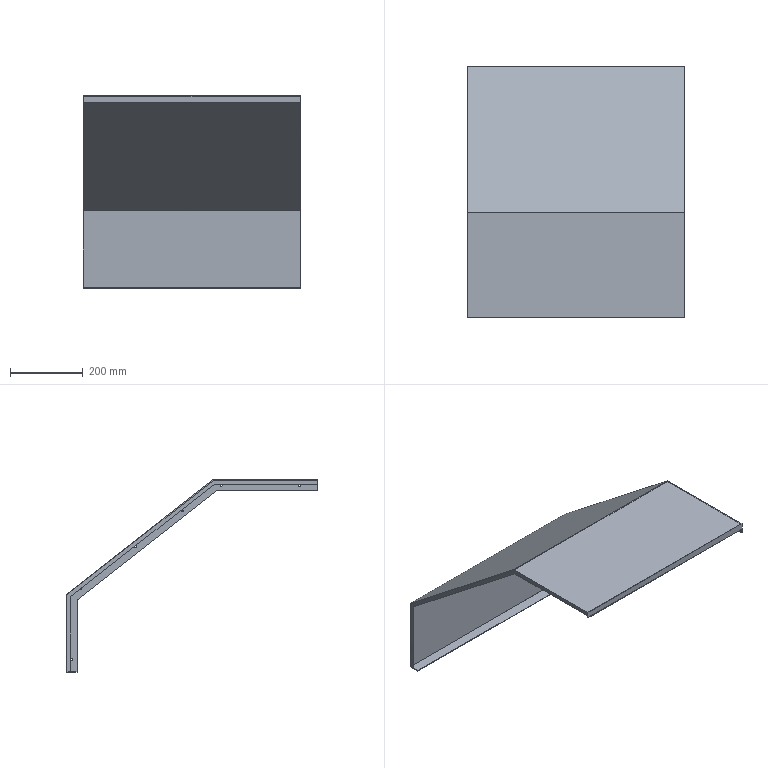Component | SolidWorks | FrontBaffle-1 | 1 solid | 33 faces | box 597 x 690 x 527.05 mm | volume 1332311 mm3 | plane 21 | cylinder 12 | commonest cylinder face diameters 6 x12
build123d program:
from build123d import *

# Parameters (mm, degrees)
EXTRUDE_THIN1_DEPTH = 595
SHELL1_T            = -2
EXTRUDE_THIN2_DEPTH = 2
SKETCH3_W           = 597
SKETCH3_H           = 2
EXTRUDE_THIN3_DEPTH = 16
SKETCH4_W           = 597
SKETCH4_H           = 30
BOSS_EXTRUDE1_DEPTH = 2
SKETCH5_R           = 3
CUT_EXTRUDE1_DEPTH  = 2


with BuildPart() as part:
    # Sketch1 → Extrude-Thin1 (new body)
    with BuildSketch(Plane.XY):
        Polygon((-90.472, -281.746), (-90.472, 6.2), (223.646, 408.252), (436.576, 408.252), (436.576, 378.252), (238.278, 378.252), (-60.472, -4.13), (-60.472, -281.746), align=None)
    extrude(amount=EXTRUDE_THIN1_DEPTH)

    # Shell1
    shell1_openings = [part.faces().sort_by_distance(p)[0] for p in [
        (88.903, 187.061, 297.5),
        (-60.472, -142.938, 297.5),
        (-75.472, -281.746, 297.5),
        (436.576, 393.252, 297.5),
        (337.427, 378.252, 297.5),
        (-81.789, -137.773, 0),
    ]]
    offset(amount=SHELL1_T, openings=shell1_openings, kind=Kind.INTERSECTION)

    # Sketch2 → Extrude-Thin2 (add)
    with BuildSketch(Plane(origin=(0, 0, 0), x_dir=(-1, 0, 0), z_dir=(0, 0, -1))):
        Polygon((-436.576, 408.252), (-223.646, 408.252), (90.472, 6.2), (90.472, -281.746), (78.472, -281.746), (78.472, 2.068), (-229.499, 396.252), (-436.576, 396.252), align=None)
    extrude(amount=EXTRUDE_THIN2_DEPTH)

    # Sketch3 → Extrude-Thin3 (add)
    with BuildSketch(Plane(origin=(-88.472, 0, 0), x_dir=(0, 0, -1), z_dir=(1, 0, 0))):
        with Locations((-296.5, -280.746)):
            Rectangle(SKETCH3_W, SKETCH3_H)
    extrude(amount=EXTRUDE_THIN3_DEPTH)

    # Sketch4 → Boss-Extrude1 (add)
    with BuildSketch(Plane(origin=(436.576, 0, 0), x_dir=(0, 0, -1), z_dir=(1, 0, 0))):
        with Locations((-296.5, 393.252)):
            Rectangle(SKETCH4_W, SKETCH4_H)
    extrude(amount=-BOSS_EXTRUDE1_DEPTH)

    # Sketch5 → Cut-Extrude1 (cut)
    with BuildSketch(Plane.XY.offset(595)):
        with Locations((-75.472, -231.746)):
            Circle(SKETCH5_R)
        with Locations((-75.472, -16.746)):
            Circle(SKETCH5_R)
        with Locations((-5.552, 90.528)):
            Circle(SKETCH5_R)
        with Locations((92.065, 217.3)):
            Circle(SKETCH5_R)
        with Locations((207.86, 367.937)):
            Circle(SKETCH5_R)
        with Locations((401.576, 393.252)):
            Circle(SKETCH5_R)
    extrude(amount=-CUT_EXTRUDE1_DEPTH, mode=Mode.SUBTRACT)


solid = part.part

# Placed as in the assembly
solid = solid.moved(Location((-889.55, -36.686, 386.009), (0, 90, 0)))
STEP:
#1=COLOUR_RGB('',0.7922,0.8196,0.9333);
#2=FILL_AREA_STYLE_COLOUR('',#1);
#3=FILL_AREA_STYLE('',(#2));
#4=SURFACE_STYLE_FILL_AREA(#3);
#5=SURFACE_SIDE_STYLE('',(#4));
#6=SURFACE_STYLE_USAGE(.BOTH.,#5);
#7=PRESENTATION_STYLE_ASSIGNMENT((#6));
#8=CARTESIAN_POINT('',(-11.675,14.038,-0.4948));
#9=VERTEX_POINT('',#8);
#10=CARTESIAN_POINT('',(-11.675,14.038,-0.731));
#11=VERTEX_POINT('',#10);
#12=CARTESIAN_POINT('',(-11.675,14.038,-0.6129));
#13=DIRECTION('',(1.,0.,-0.));
#14=DIRECTION('',(0.,0.,-1.));
#15=AXIS2_PLACEMENT_3D('',#12,#13,#14);
#16=CIRCLE('',#15,0.1181);
#17=EDGE_CURVE('',#9,#11,#16,.T.);
#18=ORIENTED_EDGE('',*,*,#17,.F.);
#19=CARTESIAN_POINT('',(-11.596,14.038,-0.4948));
#20=VERTEX_POINT('',#19);
#21=CARTESIAN_POINT('',(-11.675,14.038,-0.4948));
#22=DIRECTION('',(1.,0.,-0.));
#23=VECTOR('',#22,39.37);
#24=LINE('',#21,#23);
#25=EDGE_CURVE('',#9,#20,#24,.T.);
#26=ORIENTED_EDGE('',*,*,#25,.T.);
#27=CARTESIAN_POINT('',(-11.596,14.038,-0.731));
#28=VERTEX_POINT('',#27);
#29=CARTESIAN_POINT('',(-11.596,14.038,-0.6129));
#30=DIRECTION('',(1.,0.,-0.));
#31=DIRECTION('',(0.,0.,-1.));
#32=AXIS2_PLACEMENT_3D('',#29,#30,#31);
#33=CIRCLE('',#32,0.1181);
#34=EDGE_CURVE('',#20,#28,#33,.T.);
#35=ORIENTED_EDGE('',*,*,#34,.T.);
#36=CARTESIAN_POINT('',(-11.675,14.038,-0.731));
#37=DIRECTION('',(1.,0.,-0.));
#38=VECTOR('',#37,39.37);
#39=LINE('',#36,#38);
#40=EDGE_CURVE('',#11,#28,#39,.T.);
#41=ORIENTED_EDGE('',*,*,#40,.F.);
#42=EDGE_LOOP('',(#18,#26,#35,#41));
#43=FACE_OUTER_BOUND('',#42,.T.);
#44=CARTESIAN_POINT('',(-11.675,14.038,-0.6129));
#45=DIRECTION('',(1.,0.,-0.));
#46=DIRECTION('',(0.,0.,-1.));
#47=AXIS2_PLACEMENT_3D('',#44,#45,#46);
#48=CYLINDRICAL_SURFACE('',#47,0.1181);
#49=ADVANCED_FACE('',(#43),#48,.F.);
#50=CARTESIAN_POINT('',(-11.675,13.041,7.132));
#51=VERTEX_POINT('',#50);
#52=CARTESIAN_POINT('',(-11.675,13.041,6.896));
#53=VERTEX_POINT('',#52);
#54=CARTESIAN_POINT('',(-11.675,13.041,7.014));
#55=DIRECTION('',(1.,0.,-0.));
#56=DIRECTION('',(0.,0.,-1.));
#57=AXIS2_PLACEMENT_3D('',#54,#55,#56);
#58=CIRCLE('',#57,0.1181);
#59=EDGE_CURVE('',#51,#53,#58,.T.);
#60=ORIENTED_EDGE('',*,*,#59,.F.);
#61=CARTESIAN_POINT('',(-11.596,13.041,7.132));
#62=VERTEX_POINT('',#61);
#63=CARTESIAN_POINT('',(-11.675,13.041,7.132));
#64=DIRECTION('',(1.,0.,-0.));
#65=VECTOR('',#64,39.37);
#66=LINE('',#63,#65);
#67=EDGE_CURVE('',#51,#62,#66,.T.);
#68=ORIENTED_EDGE('',*,*,#67,.T.);
#69=CARTESIAN_POINT('',(-11.596,13.041,6.896));
#70=VERTEX_POINT('',#69);
#71=CARTESIAN_POINT('',(-11.596,13.041,7.014));
#72=DIRECTION('',(1.,0.,-0.));
#73=DIRECTION('',(0.,0.,-1.));
#74=AXIS2_PLACEMENT_3D('',#71,#72,#73);
#75=CIRCLE('',#74,0.1181);
#76=EDGE_CURVE('',#62,#70,#75,.T.);
#77=ORIENTED_EDGE('',*,*,#76,.T.);
#78=CARTESIAN_POINT('',(-11.675,13.041,6.896));
#79=DIRECTION('',(1.,0.,-0.));
#80=VECTOR('',#79,39.37);
#81=LINE('',#78,#80);
#82=EDGE_CURVE('',#53,#70,#81,.T.);
#83=ORIENTED_EDGE('',*,*,#82,.F.);
#84=EDGE_LOOP('',(#60,#68,#77,#83));
#85=FACE_OUTER_BOUND('',#84,.T.);
#86=CARTESIAN_POINT('',(-11.675,13.041,7.014));
#87=DIRECTION('',(1.,0.,-0.));
#88=DIRECTION('',(0.,0.,-1.));
#89=AXIS2_PLACEMENT_3D('',#86,#87,#88);
#90=CYLINDRICAL_SURFACE('',#89,0.1181);
#91=ADVANCED_FACE('',(#85),#90,.F.);
#92=CARTESIAN_POINT('',(-11.675,7.111,11.691));
#93=VERTEX_POINT('',#92);
#94=CARTESIAN_POINT('',(-11.675,7.111,11.455));
#95=VERTEX_POINT('',#94);
#96=CARTESIAN_POINT('',(-11.675,7.111,11.573));
#97=DIRECTION('',(1.,0.,-0.));
#98=DIRECTION('',(0.,0.,-1.));
#99=AXIS2_PLACEMENT_3D('',#96,#97,#98);
#100=CIRCLE('',#99,0.1181);
#101=EDGE_CURVE('',#93,#95,#100,.T.);
#102=ORIENTED_EDGE('',*,*,#101,.F.);
#103=CARTESIAN_POINT('',(-11.596,7.111,11.691));
#104=VERTEX_POINT('',#103);
#105=CARTESIAN_POINT('',(-11.675,7.111,11.691));
#106=DIRECTION('',(1.,0.,-0.));
#107=VECTOR('',#106,39.37);
#108=LINE('',#105,#107);
#109=EDGE_CURVE('',#93,#104,#108,.T.);
#110=ORIENTED_EDGE('',*,*,#109,.T.);
#111=CARTESIAN_POINT('',(-11.596,7.111,11.455));
#112=VERTEX_POINT('',#111);
#113=CARTESIAN_POINT('',(-11.596,7.111,11.573));
#114=DIRECTION('',(1.,0.,-0.));
#115=DIRECTION('',(0.,0.,-1.));
#116=AXIS2_PLACEMENT_3D('',#113,#114,#115);
#117=CIRCLE('',#116,0.1181);
#118=EDGE_CURVE('',#104,#112,#117,.T.);
#119=ORIENTED_EDGE('',*,*,#118,.T.);
#120=CARTESIAN_POINT('',(-11.675,7.111,11.455));
#121=DIRECTION('',(1.,0.,-0.));
#122=VECTOR('',#121,39.37);
#123=LINE('',#120,#122);
#124=EDGE_CURVE('',#95,#112,#123,.T.);
#125=ORIENTED_EDGE('',*,*,#124,.F.);
#126=EDGE_LOOP('',(#102,#110,#119,#125));
#127=FACE_OUTER_BOUND('',#126,.T.);
#128=CARTESIAN_POINT('',(-11.675,7.111,11.573));
#129=DIRECTION('',(1.,0.,-0.));
#130=DIRECTION('',(0.,0.,-1.));
#131=AXIS2_PLACEMENT_3D('',#128,#129,#130);
#132=CYLINDRICAL_SURFACE('',#131,0.1181);
#133=ADVANCED_FACE('',(#127),#132,.F.);
#134=CARTESIAN_POINT('',(-11.675,2.12,15.534));
#135=VERTEX_POINT('',#134);
#136=CARTESIAN_POINT('',(-11.675,2.12,15.298));
#137=VERTEX_POINT('',#136);
#138=CARTESIAN_POINT('',(-11.675,2.12,15.416));
#139=DIRECTION('',(1.,0.,-0.));
#140=DIRECTION('',(0.,0.,-1.));
#141=AXIS2_PLACEMENT_3D('',#138,#139,#140);
#142=CIRCLE('',#141,0.1181);
#143=EDGE_CURVE('',#135,#137,#142,.T.);
#144=ORIENTED_EDGE('',*,*,#143,.F.);
#145=CARTESIAN_POINT('',(-11.596,2.12,15.534));
#146=VERTEX_POINT('',#145);
#147=CARTESIAN_POINT('',(-11.675,2.12,15.534));
#148=DIRECTION('',(1.,0.,-0.));
#149=VECTOR('',#148,39.37);
#150=LINE('',#147,#149);
#151=EDGE_CURVE('',#135,#146,#150,.T.);
#152=ORIENTED_EDGE('',*,*,#151,.T.);
#153=CARTESIAN_POINT('',(-11.596,2.12,15.298));
#154=VERTEX_POINT('',#153);
#155=CARTESIAN_POINT('',(-11.596,2.12,15.416));
#156=DIRECTION('',(1.,0.,-0.));
#157=DIRECTION('',(0.,0.,-1.));
#158=AXIS2_PLACEMENT_3D('',#155,#156,#157);
#159=CIRCLE('',#158,0.1181);
#160=EDGE_CURVE('',#146,#154,#159,.T.);
#161=ORIENTED_EDGE('',*,*,#160,.T.);
#162=CARTESIAN_POINT('',(-11.675,2.12,15.298));
#163=DIRECTION('',(1.,0.,-0.));
#164=VECTOR('',#163,39.37);
#165=LINE('',#162,#164);
#166=EDGE_CURVE('',#137,#154,#165,.T.);
#167=ORIENTED_EDGE('',*,*,#166,.F.);
#168=EDGE_LOOP('',(#144,#152,#161,#167));
#169=FACE_OUTER_BOUND('',#168,.T.);
#170=CARTESIAN_POINT('',(-11.675,2.12,15.416));
#171=DIRECTION('',(1.,0.,-0.));
#172=DIRECTION('',(0.,0.,-1.));
#173=AXIS2_PLACEMENT_3D('',#170,#171,#172);
#174=CYLINDRICAL_SURFACE('',#173,0.1181);
#175=ADVANCED_FACE('',(#169),#174,.F.);
#176=CARTESIAN_POINT('',(-11.675,-2.104,18.287));
#177=VERTEX_POINT('',#176);
#178=CARTESIAN_POINT('',(-11.675,-2.104,18.05));
#179=VERTEX_POINT('',#178);
#180=CARTESIAN_POINT('',(-11.675,-2.104,18.169));
#181=DIRECTION('',(1.,0.,-0.));
#182=DIRECTION('',(0.,0.,-1.));
#183=AXIS2_PLACEMENT_3D('',#180,#181,#182);
#184=CIRCLE('',#183,0.1181);
#185=EDGE_CURVE('',#177,#179,#184,.T.);
#186=ORIENTED_EDGE('',*,*,#185,.F.);
#187=CARTESIAN_POINT('',(-11.596,-2.104,18.287));
#188=VERTEX_POINT('',#187);
#189=CARTESIAN_POINT('',(-11.675,-2.104,18.287));
#190=DIRECTION('',(1.,0.,-0.));
#191=VECTOR('',#190,39.37);
#192=LINE('',#189,#191);
#193=EDGE_CURVE('',#177,#188,#192,.T.);
#194=ORIENTED_EDGE('',*,*,#193,.T.);
#195=CARTESIAN_POINT('',(-11.596,-2.104,18.05));
#196=VERTEX_POINT('',#195);
#197=CARTESIAN_POINT('',(-11.596,-2.104,18.169));
#198=DIRECTION('',(1.,0.,-0.));
#199=DIRECTION('',(0.,0.,-1.));
#200=AXIS2_PLACEMENT_3D('',#197,#198,#199);
#201=CIRCLE('',#200,0.1181);
#202=EDGE_CURVE('',#188,#196,#201,.T.);
#203=ORIENTED_EDGE('',*,*,#202,.T.);
#204=CARTESIAN_POINT('',(-11.675,-2.104,18.05));
#205=DIRECTION('',(1.,0.,-0.));
#206=VECTOR('',#205,39.37);
#207=LINE('',#204,#206);
#208=EDGE_CURVE('',#179,#196,#207,.T.);
#209=ORIENTED_EDGE('',*,*,#208,.F.);
#210=EDGE_LOOP('',(#186,#194,#203,#209));
#211=FACE_OUTER_BOUND('',#210,.T.);
#212=CARTESIAN_POINT('',(-11.675,-2.104,18.169));
#213=DIRECTION('',(1.,0.,-0.));
#214=DIRECTION('',(0.,0.,-1.));
#215=AXIS2_PLACEMENT_3D('',#212,#213,#214);
#216=CYLINDRICAL_SURFACE('',#215,0.1181);
#217=ADVANCED_FACE('',(#211),#216,.F.);
#218=CARTESIAN_POINT('',(-11.675,-10.568,18.287));
#219=VERTEX_POINT('',#218);
#220=CARTESIAN_POINT('',(-11.675,-10.568,18.05));
#221=VERTEX_POINT('',#220);
#222=CARTESIAN_POINT('',(-11.675,-10.568,18.169));
#223=DIRECTION('',(1.,0.,-0.));
#224=DIRECTION('',(0.,0.,-1.));
#225=AXIS2_PLACEMENT_3D('',#222,#223,#224);
#226=CIRCLE('',#225,0.1181);
#227=EDGE_CURVE('',#219,#221,#226,.T.);
#228=ORIENTED_EDGE('',*,*,#227,.F.);
#229=CARTESIAN_POINT('',(-11.596,-10.568,18.287));
#230=VERTEX_POINT('',#229);
#231=CARTESIAN_POINT('',(-11.675,-10.568,18.287));
#232=DIRECTION('',(1.,0.,-0.));
#233=VECTOR('',#232,39.37);
#234=LINE('',#231,#233);
#235=EDGE_CURVE('',#219,#230,#234,.T.);
#236=ORIENTED_EDGE('',*,*,#235,.T.);
#237=CARTESIAN_POINT('',(-11.596,-10.568,18.05));
#238=VERTEX_POINT('',#237);
#239=CARTESIAN_POINT('',(-11.596,-10.568,18.169));
#240=DIRECTION('',(1.,0.,-0.));
#241=DIRECTION('',(0.,0.,-1.));
#242=AXIS2_PLACEMENT_3D('',#239,#240,#241);
#243=CIRCLE('',#242,0.1181);
#244=EDGE_CURVE('',#230,#238,#243,.T.);
#245=ORIENTED_EDGE('',*,*,#244,.T.);
#246=CARTESIAN_POINT('',(-11.675,-10.568,18.05));
#247=DIRECTION('',(1.,0.,-0.));
#248=VECTOR('',#247,39.37);
#249=LINE('',#246,#248);
#250=EDGE_CURVE('',#221,#238,#249,.T.);
#251=ORIENTED_EDGE('',*,*,#250,.F.);
#252=EDGE_LOOP('',(#228,#236,#245,#251));
#253=FACE_OUTER_BOUND('',#252,.T.);
#254=CARTESIAN_POINT('',(-11.675,-10.568,18.169));
#255=DIRECTION('',(1.,0.,-0.));
#256=DIRECTION('',(0.,0.,-1.));
#257=AXIS2_PLACEMENT_3D('',#254,#255,#256);
#258=CYLINDRICAL_SURFACE('',#257,0.1181);
#259=ADVANCED_FACE('',(#253),#258,.F.);
#260=CARTESIAN_POINT('',(-11.675,14.55,-1.912));
#261=VERTEX_POINT('',#260);
#262=CARTESIAN_POINT('',(-35.022,14.55,-1.912));
#263=VERTEX_POINT('',#262);
#264=CARTESIAN_POINT('',(-11.596,14.55,-1.912));
#265=DIRECTION('',(-1.,-0.,0.));
#266=VECTOR('',#265,39.37);
#267=LINE('',#264,#266);
#268=EDGE_CURVE('',#261,#263,#267,.T.);
#269=ORIENTED_EDGE('',*,*,#268,.F.);
#270=CARTESIAN_POINT('',(-11.675,14.55,6.354));
#271=VERTEX_POINT('',#270);
#272=CARTESIAN_POINT('',(-11.675,14.55,15.197));
#273=DIRECTION('',(-0.,-0.,-1.));
#274=VECTOR('',#273,39.37);
#275=LINE('',#272,#274);
#276=EDGE_CURVE('',#271,#261,#275,.T.);
#277=ORIENTED_EDGE('',*,*,#276,.F.);
#278=CARTESIAN_POINT('',(-35.022,14.55,6.354));
#279=VERTEX_POINT('',#278);
#280=CARTESIAN_POINT('',(-11.596,14.55,6.354));
#281=DIRECTION('',(-1.,-0.,0.));
#282=VECTOR('',#281,39.37);
#283=LINE('',#280,#282);
#284=EDGE_CURVE('',#271,#279,#283,.T.);
#285=ORIENTED_EDGE('',*,*,#284,.T.);
#286=CARTESIAN_POINT('',(-35.022,14.55,15.197));
#287=DIRECTION('',(-0.,-0.,-1.));
#288=VECTOR('',#287,39.37);
#289=LINE('',#286,#288);
#290=EDGE_CURVE('',#279,#263,#289,.T.);
#291=ORIENTED_EDGE('',*,*,#290,.T.);
#292=EDGE_LOOP('',(#269,#277,#285,#291));
#293=FACE_OUTER_BOUND('',#292,.T.);
#294=CARTESIAN_POINT('',(-11.596,14.55,6.392));
#295=DIRECTION('',(-0.,1.,-0.));
#296=DIRECTION('',(0.,0.,1.));
#297=AXIS2_PLACEMENT_3D('',#294,#295,#296);
#298=PLANE('',#297);
#299=ADVANCED_FACE('',(#293),#298,.F.);
#300=CARTESIAN_POINT('',(-11.675,14.038,-0.6129));
#301=DIRECTION('',(1.,0.,-0.));
#302=DIRECTION('',(0.,0.,-1.));
#303=AXIS2_PLACEMENT_3D('',#300,#301,#302);
#304=CIRCLE('',#303,0.1181);
#305=EDGE_CURVE('',#11,#9,#304,.T.);
#306=ORIENTED_EDGE('',*,*,#305,.T.);
#307=ORIENTED_EDGE('',*,*,#17,.T.);
#308=EDGE_LOOP('',(#306,#307));
#309=FACE_BOUND('',#308,.T.);
#310=CARTESIAN_POINT('',(-11.675,13.041,7.014));
#311=DIRECTION('',(1.,0.,-0.));
#312=DIRECTION('',(0.,0.,-1.));
#313=AXIS2_PLACEMENT_3D('',#310,#311,#312);
#314=CIRCLE('',#313,0.1181);
#315=EDGE_CURVE('',#53,#51,#314,.T.);
#316=ORIENTED_EDGE('',*,*,#315,.T.);
#317=ORIENTED_EDGE('',*,*,#59,.T.);
#318=EDGE_LOOP('',(#316,#317));
#319=FACE_BOUND('',#318,.T.);
#320=CARTESIAN_POINT('',(-11.675,7.111,11.573));
#321=DIRECTION('',(1.,0.,-0.));
#322=DIRECTION('',(0.,0.,-1.));
#323=AXIS2_PLACEMENT_3D('',#320,#321,#322);
#324=CIRCLE('',#323,0.1181);
#325=EDGE_CURVE('',#95,#93,#324,.T.);
#326=ORIENTED_EDGE('',*,*,#325,.T.);
#327=ORIENTED_EDGE('',*,*,#101,.T.);
#328=EDGE_LOOP('',(#326,#327));
#329=FACE_BOUND('',#328,.T.);
#330=CARTESIAN_POINT('',(-11.675,2.12,15.416));
#331=DIRECTION('',(1.,0.,-0.));
#332=DIRECTION('',(0.,0.,-1.));
#333=AXIS2_PLACEMENT_3D('',#330,#331,#332);
#334=CIRCLE('',#333,0.1181);
#335=EDGE_CURVE('',#137,#135,#334,.T.);
#336=ORIENTED_EDGE('',*,*,#335,.T.);
#337=ORIENTED_EDGE('',*,*,#143,.T.);
#338=EDGE_LOOP('',(#336,#337));
#339=FACE_BOUND('',#338,.T.);
#340=CARTESIAN_POINT('',(-11.675,-2.104,18.169));
#341=DIRECTION('',(1.,0.,-0.));
#342=DIRECTION('',(0.,0.,-1.));
#343=AXIS2_PLACEMENT_3D('',#340,#341,#342);
#344=CIRCLE('',#343,0.1181);
#345=EDGE_CURVE('',#179,#177,#344,.T.);
#346=ORIENTED_EDGE('',*,*,#345,.T.);
#347=ORIENTED_EDGE('',*,*,#185,.T.);
#348=EDGE_LOOP('',(#346,#347));
#349=FACE_BOUND('',#348,.T.);
#350=CARTESIAN_POINT('',(-11.675,-10.568,18.169));
#351=DIRECTION('',(1.,0.,-0.));
#352=DIRECTION('',(0.,0.,-1.));
#353=AXIS2_PLACEMENT_3D('',#350,#351,#352);
#354=CIRCLE('',#353,0.1181);
#355=EDGE_CURVE('',#221,#219,#354,.T.);
#356=ORIENTED_EDGE('',*,*,#355,.T.);
#357=ORIENTED_EDGE('',*,*,#227,.T.);
#358=EDGE_LOOP('',(#356,#357));
#359=FACE_BOUND('',#358,.T.);
#360=ORIENTED_EDGE('',*,*,#276,.T.);
#361=CARTESIAN_POINT('',(-11.675,13.447,-1.912));
#362=VERTEX_POINT('',#361);
#363=CARTESIAN_POINT('',(-11.675,-1.444,-1.912));
#364=DIRECTION('',(0.,-1.,0.));
#365=VECTOR('',#364,39.37);
#366=LINE('',#363,#365);
#367=EDGE_CURVE('',#261,#362,#366,.T.);
#368=ORIENTED_EDGE('',*,*,#367,.T.);
#369=CARTESIAN_POINT('',(-11.675,13.447,5.816));
#370=VERTEX_POINT('',#369);
#371=CARTESIAN_POINT('',(-11.675,13.447,15.197));
#372=DIRECTION('',(-0.,-0.,-1.));
#373=VECTOR('',#372,39.37);
#374=LINE('',#371,#373);
#375=EDGE_CURVE('',#370,#362,#374,.T.);
#376=ORIENTED_EDGE('',*,*,#375,.F.);
#377=CARTESIAN_POINT('',(-11.675,-1.607,17.578));
#378=VERTEX_POINT('',#377);
#379=CARTESIAN_POINT('',(-11.675,-0.3509,16.597));
#380=DIRECTION('',(-0.,0.788,-0.6157));
#381=VECTOR('',#380,39.37);
#382=LINE('',#379,#381);
#383=EDGE_CURVE('',#378,#370,#382,.T.);
#384=ORIENTED_EDGE('',*,*,#383,.F.);
#385=CARTESIAN_POINT('',(-11.675,-12.537,17.578));
#386=VERTEX_POINT('',#385);
#387=CARTESIAN_POINT('',(-11.675,-1.444,17.578));
#388=DIRECTION('',(-0.,1.,-0.));
#389=VECTOR('',#388,39.37);
#390=LINE('',#387,#389);
#391=EDGE_CURVE('',#386,#378,#390,.T.);
#392=ORIENTED_EDGE('',*,*,#391,.F.);
#393=CARTESIAN_POINT('',(-11.675,-12.537,18.05));
#394=VERTEX_POINT('',#393);
#395=CARTESIAN_POINT('',(-11.675,-12.537,15.197));
#396=DIRECTION('',(0.,0.,1.));
#397=VECTOR('',#396,39.37);
#398=LINE('',#395,#397);
#399=EDGE_CURVE('',#386,#394,#398,.T.);
#400=ORIENTED_EDGE('',*,*,#399,.T.);
#401=CARTESIAN_POINT('',(-11.675,-12.458,18.05));
#402=VERTEX_POINT('',#401);
#403=CARTESIAN_POINT('',(-11.675,-1.444,18.05));
#404=DIRECTION('',(-0.,1.,-0.));
#405=VECTOR('',#404,39.37);
#406=LINE('',#403,#405);
#407=EDGE_CURVE('',#394,#402,#406,.T.);
#408=ORIENTED_EDGE('',*,*,#407,.T.);
#409=CARTESIAN_POINT('',(-11.675,-12.458,18.68));
#410=VERTEX_POINT('',#409);
#411=CARTESIAN_POINT('',(-11.675,-12.458,15.197));
#412=DIRECTION('',(-0.,-0.,-1.));
#413=VECTOR('',#412,39.37);
#414=LINE('',#411,#413);
#415=EDGE_CURVE('',#410,#402,#414,.T.);
#416=ORIENTED_EDGE('',*,*,#415,.F.);
#417=CARTESIAN_POINT('',(-11.675,-1.227,18.68));
#418=VERTEX_POINT('',#417);
#419=CARTESIAN_POINT('',(-11.675,-1.444,18.68));
#420=DIRECTION('',(-0.,1.,-0.));
#421=VECTOR('',#420,39.37);
#422=LINE('',#419,#421);
#423=EDGE_CURVE('',#410,#418,#422,.T.);
#424=ORIENTED_EDGE('',*,*,#423,.T.);
#425=CARTESIAN_POINT('',(-11.675,0.3277,17.465));
#426=DIRECTION('',(-0.,0.788,-0.6157));
#427=VECTOR('',#426,39.37);
#428=LINE('',#425,#427);
#429=EDGE_CURVE('',#418,#271,#428,.T.);
#430=ORIENTED_EDGE('',*,*,#429,.T.);
#431=EDGE_LOOP('',(#360,#368,#376,#384,#392,#400,#408,#416,#424,#430));
#432=FACE_OUTER_BOUND('',#431,.T.);
#433=CARTESIAN_POINT('',(-11.675,-1.444,15.197));
#434=DIRECTION('',(-1.,-0.,0.));
#435=DIRECTION('',(0.,0.,1.));
#436=AXIS2_PLACEMENT_3D('',#433,#434,#435);
#437=PLANE('',#436);
#438=ADVANCED_FACE('',(#309,#319,#329,#339,#349,#359,#432),#437,.T.);
#439=CARTESIAN_POINT('',(-35.022,14.156,-1.912));
#440=VERTEX_POINT('',#439);
#441=CARTESIAN_POINT('',(-35.1,14.156,-1.912));
#442=VERTEX_POINT('',#441);
#443=CARTESIAN_POINT('',(-35.1,14.156,-1.912));
#444=DIRECTION('',(-1.,-0.,0.));
#445=VECTOR('',#444,39.37);
#446=LINE('',#443,#445);
#447=EDGE_CURVE('',#440,#442,#446,.T.);
#448=ORIENTED_EDGE('',*,*,#447,.F.);
#449=CARTESIAN_POINT('',(-35.022,14.156,6.162));
#450=VERTEX_POINT('',#449);
#451=CARTESIAN_POINT('',(-35.022,14.156,-1.991));
#452=DIRECTION('',(0.,0.,1.));
#453=VECTOR('',#452,39.37);
#454=LINE('',#451,#453);
#455=EDGE_CURVE('',#440,#450,#454,.T.);
#456=ORIENTED_EDGE('',*,*,#455,.T.);
#457=CARTESIAN_POINT('',(-35.1,14.156,6.162));
#458=VERTEX_POINT('',#457);
#459=CARTESIAN_POINT('',(-35.1,14.156,6.162));
#460=DIRECTION('',(1.,0.,-0.));
#461=VECTOR('',#460,39.37);
#462=LINE('',#459,#461);
#463=EDGE_CURVE('',#458,#450,#462,.T.);
#464=ORIENTED_EDGE('',*,*,#463,.F.);
#465=CARTESIAN_POINT('',(-35.1,14.156,-1.991));
#466=DIRECTION('',(0.,0.,1.));
#467=VECTOR('',#466,39.37);
#468=LINE('',#465,#467);
#469=EDGE_CURVE('',#442,#458,#468,.T.);
#470=ORIENTED_EDGE('',*,*,#469,.F.);
#471=EDGE_LOOP('',(#448,#456,#464,#470));
#472=FACE_OUTER_BOUND('',#471,.T.);
#473=CARTESIAN_POINT('',(-35.1,14.156,-1.991));
#474=DIRECTION('',(-0.,1.,-0.));
#475=DIRECTION('',(0.,0.,1.));
#476=AXIS2_PLACEMENT_3D('',#473,#474,#475);
#477=PLANE('',#476);
#478=ADVANCED_FACE('',(#472),#477,.F.);
#479=CARTESIAN_POINT('',(-35.022,-1.444,-1.912));
#480=DIRECTION('',(0.,-1.,0.));
#481=VECTOR('',#480,39.37);
#482=LINE('',#479,#481);
#483=EDGE_CURVE('',#263,#440,#482,.T.);
#484=ORIENTED_EDGE('',*,*,#483,.F.);
#485=ORIENTED_EDGE('',*,*,#290,.F.);
#486=CARTESIAN_POINT('',(-35.022,-1.227,18.68));
#487=VERTEX_POINT('',#486);
#488=CARTESIAN_POINT('',(-35.022,0.3277,17.465));
#489=DIRECTION('',(-0.,0.788,-0.6157));
#490=VECTOR('',#489,39.37);
#491=LINE('',#488,#490);
#492=EDGE_CURVE('',#487,#279,#491,.T.);
#493=ORIENTED_EDGE('',*,*,#492,.F.);
#494=CARTESIAN_POINT('',(-35.022,-12.458,18.68));
#495=VERTEX_POINT('',#494);
#496=CARTESIAN_POINT('',(-35.022,-1.444,18.68));
#497=DIRECTION('',(-0.,1.,-0.));
#498=VECTOR('',#497,39.37);
#499=LINE('',#496,#498);
#500=EDGE_CURVE('',#495,#487,#499,.T.);
#501=ORIENTED_EDGE('',*,*,#500,.F.);
#502=CARTESIAN_POINT('',(-35.022,-12.458,18.287));
#503=VERTEX_POINT('',#502);
#504=CARTESIAN_POINT('',(-35.022,-12.458,15.197));
#505=DIRECTION('',(-0.,-0.,-1.));
#506=VECTOR('',#505,39.37);
#507=LINE('',#504,#506);
#508=EDGE_CURVE('',#495,#503,#507,.T.);
#509=ORIENTED_EDGE('',*,*,#508,.T.);
#510=CARTESIAN_POINT('',(-35.022,-1.363,18.287));
#511=VERTEX_POINT('',#510);
#512=CARTESIAN_POINT('',(-35.022,-1.2,18.287));
#513=DIRECTION('',(0.,-1.,0.));
#514=VECTOR('',#513,39.37);
#515=LINE('',#512,#514);
#516=EDGE_CURVE('',#511,#503,#515,.T.);
#517=ORIENTED_EDGE('',*,*,#516,.F.);
#518=CARTESIAN_POINT('',(-35.022,14.338,6.02));
#519=DIRECTION('',(0.,-0.788,0.6157));
#520=VECTOR('',#519,39.37);
#521=LINE('',#518,#520);
#522=EDGE_CURVE('',#450,#511,#521,.T.);
#523=ORIENTED_EDGE('',*,*,#522,.F.);
#524=ORIENTED_EDGE('',*,*,#455,.F.);
#525=EDGE_LOOP('',(#484,#485,#493,#501,#509,#517,#523,#524));
#526=FACE_OUTER_BOUND('',#525,.T.);
#527=CARTESIAN_POINT('',(-35.022,-1.444,15.197));
#528=DIRECTION('',(-1.,-0.,0.));
#529=DIRECTION('',(0.,0.,1.));
#530=AXIS2_PLACEMENT_3D('',#527,#528,#529);
#531=PLANE('',#530);
#532=ADVANCED_FACE('',(#526),#531,.F.);
#533=CARTESIAN_POINT('',(-11.596,13.447,-1.991));
#534=VERTEX_POINT('',#533);
#535=CARTESIAN_POINT('',(-35.1,13.447,-1.991));
#536=VERTEX_POINT('',#535);
#537=CARTESIAN_POINT('',(-11.596,13.447,-1.991));
#538=DIRECTION('',(-1.,-0.,0.));
#539=VECTOR('',#538,39.37);
#540=LINE('',#537,#539);
#541=EDGE_CURVE('',#534,#536,#540,.T.);
#542=ORIENTED_EDGE('',*,*,#541,.T.);
#543=CARTESIAN_POINT('',(-35.1,14.629,-1.991));
#544=VERTEX_POINT('',#543);
#545=CARTESIAN_POINT('',(-35.1,14.156,-1.991));
#546=DIRECTION('',(-0.,1.,-0.));
#547=VECTOR('',#546,39.37);
#548=LINE('',#545,#547);
#549=EDGE_CURVE('',#536,#544,#548,.T.);
#550=ORIENTED_EDGE('',*,*,#549,.T.);
#551=CARTESIAN_POINT('',(-11.596,14.629,-1.991));
#552=VERTEX_POINT('',#551);
#553=CARTESIAN_POINT('',(-11.596,14.629,-1.991));
#554=DIRECTION('',(-1.,-0.,0.));
#555=VECTOR('',#554,39.37);
#556=LINE('',#553,#555);
#557=EDGE_CURVE('',#552,#544,#556,.T.);
#558=ORIENTED_EDGE('',*,*,#557,.F.);
#559=CARTESIAN_POINT('',(-11.596,14.629,-1.991));
#560=DIRECTION('',(0.,-1.,0.));
#561=VECTOR('',#560,39.37);
#562=LINE('',#559,#561);
#563=EDGE_CURVE('',#552,#534,#562,.T.);
#564=ORIENTED_EDGE('',*,*,#563,.T.);
#565=EDGE_LOOP('',(#542,#550,#558,#564));
#566=FACE_OUTER_BOUND('',#565,.T.);
#567=CARTESIAN_POINT('',(-11.596,14.629,-1.991));
#568=DIRECTION('',(-0.,-0.,-1.));
#569=DIRECTION('',(-1.,-0.,0.));
#570=AXIS2_PLACEMENT_3D('',#567,#568,#569);
#571=PLANE('',#570);
#572=ADVANCED_FACE('',(#566),#571,.T.);
#573=ORIENTED_EDGE('',*,*,#541,.F.);
#574=CARTESIAN_POINT('',(-11.596,13.447,5.816));
#575=VERTEX_POINT('',#574);
#576=CARTESIAN_POINT('',(-11.596,13.447,6.392));
#577=DIRECTION('',(-0.,-0.,-1.));
#578=VECTOR('',#577,39.37);
#579=LINE('',#576,#578);
#580=EDGE_CURVE('',#575,#534,#579,.T.);
#581=ORIENTED_EDGE('',*,*,#580,.F.);
#582=CARTESIAN_POINT('',(-11.596,13.447,5.816));
#583=DIRECTION('',(-1.,-0.,0.));
#584=VECTOR('',#583,39.37);
#585=LINE('',#582,#584);
#586=EDGE_CURVE('',#575,#370,#585,.T.);
#587=ORIENTED_EDGE('',*,*,#586,.T.);
#588=ORIENTED_EDGE('',*,*,#375,.T.);
#589=CARTESIAN_POINT('',(-35.1,13.447,-1.912));
#590=VERTEX_POINT('',#589);
#591=CARTESIAN_POINT('',(-11.596,13.447,-1.912));
#592=DIRECTION('',(-1.,-0.,0.));
#593=VECTOR('',#592,39.37);
#594=LINE('',#591,#593);
#595=EDGE_CURVE('',#362,#590,#594,.T.);
#596=ORIENTED_EDGE('',*,*,#595,.T.);
#597=CARTESIAN_POINT('',(-35.1,13.447,-1.912));
#598=DIRECTION('',(-0.,-0.,-1.));
#599=VECTOR('',#598,39.37);
#600=LINE('',#597,#599);
#601=EDGE_CURVE('',#590,#536,#600,.T.);
#602=ORIENTED_EDGE('',*,*,#601,.T.);
#603=EDGE_LOOP('',(#573,#581,#587,#588,#596,#602));
#604=FACE_OUTER_BOUND('',#603,.T.);
#605=CARTESIAN_POINT('',(-11.596,13.447,6.392));
#606=DIRECTION('',(-0.,1.,-0.));
#607=DIRECTION('',(0.,0.,1.));
#608=AXIS2_PLACEMENT_3D('',#605,#606,#607);
#609=PLANE('',#608);
#610=ADVANCED_FACE('',(#604),#609,.F.);
#611=CARTESIAN_POINT('',(-35.1,14.629,6.392));
#612=VERTEX_POINT('',#611);
#613=CARTESIAN_POINT('',(-35.1,14.629,-1.991));
#614=DIRECTION('',(0.,0.,1.));
#615=VECTOR('',#614,39.37);
#616=LINE('',#613,#615);
#617=EDGE_CURVE('',#544,#612,#616,.T.);
#618=ORIENTED_EDGE('',*,*,#617,.T.);
#619=CARTESIAN_POINT('',(-11.596,14.629,6.392));
#620=VERTEX_POINT('',#619);
#621=CARTESIAN_POINT('',(-11.596,14.629,6.392));
#622=DIRECTION('',(-1.,-0.,0.));
#623=VECTOR('',#622,39.37);
#624=LINE('',#621,#623);
#625=EDGE_CURVE('',#620,#612,#624,.T.);
#626=ORIENTED_EDGE('',*,*,#625,.F.);
#627=CARTESIAN_POINT('',(-11.596,14.629,6.392));
#628=DIRECTION('',(-0.,-0.,-1.));
#629=VECTOR('',#628,39.37);
#630=LINE('',#627,#629);
#631=EDGE_CURVE('',#620,#552,#630,.T.);
#632=ORIENTED_EDGE('',*,*,#631,.T.);
#633=ORIENTED_EDGE('',*,*,#557,.T.);
#634=EDGE_LOOP('',(#618,#626,#632,#633));
#635=FACE_OUTER_BOUND('',#634,.T.);
#636=CARTESIAN_POINT('',(-11.596,14.629,6.392));
#637=DIRECTION('',(-0.,1.,-0.));
#638=DIRECTION('',(0.,0.,1.));
#639=AXIS2_PLACEMENT_3D('',#636,#637,#638);
#640=PLANE('',#639);
#641=ADVANCED_FACE('',(#635),#640,.T.);
#642=ORIENTED_EDGE('',*,*,#625,.T.);
#643=CARTESIAN_POINT('',(-35.1,-1.2,18.759));
#644=VERTEX_POINT('',#643);
#645=CARTESIAN_POINT('',(-35.1,14.629,6.392));
#646=DIRECTION('',(0.,-0.788,0.6157));
#647=VECTOR('',#646,39.37);
#648=LINE('',#645,#647);
#649=EDGE_CURVE('',#612,#644,#648,.T.);
#650=ORIENTED_EDGE('',*,*,#649,.T.);
#651=CARTESIAN_POINT('',(-11.596,-1.2,18.759));
#652=VERTEX_POINT('',#651);
#653=CARTESIAN_POINT('',(-11.596,-1.2,18.759));
#654=DIRECTION('',(-1.,-0.,0.));
#655=VECTOR('',#654,39.37);
#656=LINE('',#653,#655);
#657=EDGE_CURVE('',#652,#644,#656,.T.);
#658=ORIENTED_EDGE('',*,*,#657,.F.);
#659=CARTESIAN_POINT('',(-11.596,-1.2,18.759));
#660=DIRECTION('',(-0.,0.788,-0.6157));
#661=VECTOR('',#660,39.37);
#662=LINE('',#659,#661);
#663=EDGE_CURVE('',#652,#620,#662,.T.);
#664=ORIENTED_EDGE('',*,*,#663,.T.);
#665=EDGE_LOOP('',(#642,#650,#658,#664));
#666=FACE_OUTER_BOUND('',#665,.T.);
#667=CARTESIAN_POINT('',(-11.596,-1.2,18.759));
#668=DIRECTION('',(-0.,0.6157,0.788));
#669=DIRECTION('',(0.,-0.788,0.6157));
#670=AXIS2_PLACEMENT_3D('',#667,#668,#669);
#671=PLANE('',#670);
#672=ADVANCED_FACE('',(#666),#671,.T.);
#673=ORIENTED_EDGE('',*,*,#657,.T.);
#674=CARTESIAN_POINT('',(-35.1,-12.537,18.759));
#675=VERTEX_POINT('',#674);
#676=CARTESIAN_POINT('',(-35.1,-1.2,18.759));
#677=DIRECTION('',(0.,-1.,0.));
#678=VECTOR('',#677,39.37);
#679=LINE('',#676,#678);
#680=EDGE_CURVE('',#644,#675,#679,.T.);
#681=ORIENTED_EDGE('',*,*,#680,.T.);
#682=CARTESIAN_POINT('',(-11.596,-12.537,18.759));
#683=VERTEX_POINT('',#682);
#684=CARTESIAN_POINT('',(-11.596,-12.537,18.759));
#685=DIRECTION('',(-1.,-0.,0.));
#686=VECTOR('',#685,39.37);
#687=LINE('',#684,#686);
#688=EDGE_CURVE('',#683,#675,#687,.T.);
#689=ORIENTED_EDGE('',*,*,#688,.F.);
#690=CARTESIAN_POINT('',(-11.596,-12.537,18.759));
#691=DIRECTION('',(-0.,1.,-0.));
#692=VECTOR('',#691,39.37);
#693=LINE('',#690,#692);
#694=EDGE_CURVE('',#683,#652,#693,.T.);
#695=ORIENTED_EDGE('',*,*,#694,.T.);
#696=EDGE_LOOP('',(#673,#681,#689,#695));
#697=FACE_OUTER_BOUND('',#696,.T.);
#698=CARTESIAN_POINT('',(-11.596,-12.537,18.759));
#699=DIRECTION('',(0.,0.,1.));
#700=DIRECTION('',(1.,0.,-0.));
#701=AXIS2_PLACEMENT_3D('',#698,#699,#700);
#702=PLANE('',#701);
#703=ADVANCED_FACE('',(#697),#702,.T.);
#704=CARTESIAN_POINT('',(-35.1,-12.537,18.05));
#705=VERTEX_POINT('',#704);
#706=CARTESIAN_POINT('',(-35.1,-12.537,18.759));
#707=DIRECTION('',(-0.,-0.,-1.));
#708=VECTOR('',#707,39.37);
#709=LINE('',#706,#708);
#710=EDGE_CURVE('',#675,#705,#709,.T.);
#711=ORIENTED_EDGE('',*,*,#710,.T.);
#712=CARTESIAN_POINT('',(-11.596,-12.537,18.05));
#713=DIRECTION('',(-1.,-0.,0.));
#714=VECTOR('',#713,39.37);
#715=LINE('',#712,#714);
#716=EDGE_CURVE('',#394,#705,#715,.T.);
#717=ORIENTED_EDGE('',*,*,#716,.F.);
#718=ORIENTED_EDGE('',*,*,#399,.F.);
#719=CARTESIAN_POINT('',(-11.596,-12.537,17.578));
#720=VERTEX_POINT('',#719);
#721=CARTESIAN_POINT('',(-11.596,-12.537,17.578));
#722=DIRECTION('',(-1.,-0.,0.));
#723=VECTOR('',#722,39.37);
#724=LINE('',#721,#723);
#725=EDGE_CURVE('',#720,#386,#724,.T.);
#726=ORIENTED_EDGE('',*,*,#725,.F.);
#727=CARTESIAN_POINT('',(-11.596,-12.537,17.578));
#728=DIRECTION('',(0.,0.,1.));
#729=VECTOR('',#728,39.37);
#730=LINE('',#727,#729);
#731=EDGE_CURVE('',#720,#683,#730,.T.);
#732=ORIENTED_EDGE('',*,*,#731,.T.);
#733=ORIENTED_EDGE('',*,*,#688,.T.);
#734=EDGE_LOOP('',(#711,#717,#718,#726,#732,#733));
#735=FACE_OUTER_BOUND('',#734,.T.);
#736=CARTESIAN_POINT('',(-11.596,-12.537,17.578));
#737=DIRECTION('',(0.,-1.,0.));
#738=DIRECTION('',(-1.,-0.,0.));
#739=AXIS2_PLACEMENT_3D('',#736,#737,#738);
#740=PLANE('',#739);
#741=ADVANCED_FACE('',(#735),#740,.T.);
#742=ORIENTED_EDGE('',*,*,#725,.T.);
#743=ORIENTED_EDGE('',*,*,#391,.T.);
#744=CARTESIAN_POINT('',(-11.596,-1.607,17.578));
#745=VERTEX_POINT('',#744);
#746=CARTESIAN_POINT('',(-11.596,-1.607,17.578));
#747=DIRECTION('',(-1.,-0.,0.));
#748=VECTOR('',#747,39.37);
#749=LINE('',#746,#748);
#750=EDGE_CURVE('',#745,#378,#749,.T.);
#751=ORIENTED_EDGE('',*,*,#750,.F.);
#752=CARTESIAN_POINT('',(-11.596,-12.537,17.578));
#753=DIRECTION('',(-0.,1.,-0.));
#754=VECTOR('',#753,39.37);
#755=LINE('',#752,#754);
#756=EDGE_CURVE('',#720,#745,#755,.T.);
#757=ORIENTED_EDGE('',*,*,#756,.F.);
#758=EDGE_LOOP('',(#742,#743,#751,#757));
#759=FACE_OUTER_BOUND('',#758,.T.);
#760=CARTESIAN_POINT('',(-11.596,-12.537,17.578));
#761=DIRECTION('',(0.,0.,1.));
#762=DIRECTION('',(1.,0.,-0.));
#763=AXIS2_PLACEMENT_3D('',#760,#761,#762);
#764=PLANE('',#763);
#765=ADVANCED_FACE('',(#759),#764,.F.);
#766=ORIENTED_EDGE('',*,*,#750,.T.);
#767=ORIENTED_EDGE('',*,*,#383,.T.);
#768=ORIENTED_EDGE('',*,*,#586,.F.);
#769=CARTESIAN_POINT('',(-11.596,-1.927,17.828));
#770=DIRECTION('',(-0.,0.788,-0.6157));
#771=VECTOR('',#770,39.37);
#772=LINE('',#769,#771);
#773=EDGE_CURVE('',#745,#575,#772,.T.);
#774=ORIENTED_EDGE('',*,*,#773,.F.);
#775=EDGE_LOOP('',(#766,#767,#768,#774));
#776=FACE_OUTER_BOUND('',#775,.T.);
#777=CARTESIAN_POINT('',(-11.596,-1.927,17.828));
#778=DIRECTION('',(-0.,0.6157,0.788));
#779=DIRECTION('',(0.,-0.788,0.6157));
#780=AXIS2_PLACEMENT_3D('',#777,#778,#779);
#781=PLANE('',#780);
#782=ADVANCED_FACE('',(#776),#781,.F.);
#783=CARTESIAN_POINT('',(-11.596,14.038,-0.6129));
#784=DIRECTION('',(1.,0.,-0.));
#785=DIRECTION('',(0.,0.,-1.));
#786=AXIS2_PLACEMENT_3D('',#783,#784,#785);
#787=CIRCLE('',#786,0.1181);
#788=EDGE_CURVE('',#28,#20,#787,.T.);
#789=ORIENTED_EDGE('',*,*,#788,.F.);
#790=ORIENTED_EDGE('',*,*,#34,.F.);
#791=EDGE_LOOP('',(#789,#790));
#792=FACE_BOUND('',#791,.T.);
#793=CARTESIAN_POINT('',(-11.596,13.041,7.014));
#794=DIRECTION('',(1.,0.,-0.));
#795=DIRECTION('',(0.,0.,-1.));
#796=AXIS2_PLACEMENT_3D('',#793,#794,#795);
#797=CIRCLE('',#796,0.1181);
#798=EDGE_CURVE('',#70,#62,#797,.T.);
#799=ORIENTED_EDGE('',*,*,#798,.F.);
#800=ORIENTED_EDGE('',*,*,#76,.F.);
#801=EDGE_LOOP('',(#799,#800));
#802=FACE_BOUND('',#801,.T.);
#803=CARTESIAN_POINT('',(-11.596,7.111,11.573));
#804=DIRECTION('',(1.,0.,-0.));
#805=DIRECTION('',(0.,0.,-1.));
#806=AXIS2_PLACEMENT_3D('',#803,#804,#805);
#807=CIRCLE('',#806,0.1181);
#808=EDGE_CURVE('',#112,#104,#807,.T.);
#809=ORIENTED_EDGE('',*,*,#808,.F.);
#810=ORIENTED_EDGE('',*,*,#118,.F.);
#811=EDGE_LOOP('',(#809,#810));
#812=FACE_BOUND('',#811,.T.);
#813=CARTESIAN_POINT('',(-11.596,2.12,15.416));
#814=DIRECTION('',(1.,0.,-0.));
#815=DIRECTION('',(0.,0.,-1.));
#816=AXIS2_PLACEMENT_3D('',#813,#814,#815);
#817=CIRCLE('',#816,0.1181);
#818=EDGE_CURVE('',#154,#146,#817,.T.);
#819=ORIENTED_EDGE('',*,*,#818,.F.);
#820=ORIENTED_EDGE('',*,*,#160,.F.);
#821=EDGE_LOOP('',(#819,#820));
#822=FACE_BOUND('',#821,.T.);
#823=CARTESIAN_POINT('',(-11.596,-2.104,18.169));
#824=DIRECTION('',(1.,0.,-0.));
#825=DIRECTION('',(0.,0.,-1.));
#826=AXIS2_PLACEMENT_3D('',#823,#824,#825);
#827=CIRCLE('',#826,0.1181);
#828=EDGE_CURVE('',#196,#188,#827,.T.);
#829=ORIENTED_EDGE('',*,*,#828,.F.);
#830=ORIENTED_EDGE('',*,*,#202,.F.);
#831=EDGE_LOOP('',(#829,#830));
#832=FACE_BOUND('',#831,.T.);
#833=CARTESIAN_POINT('',(-11.596,-10.568,18.169));
#834=DIRECTION('',(1.,0.,-0.));
#835=DIRECTION('',(0.,0.,-1.));
#836=AXIS2_PLACEMENT_3D('',#833,#834,#835);
#837=CIRCLE('',#836,0.1181);
#838=EDGE_CURVE('',#238,#230,#837,.T.);
#839=ORIENTED_EDGE('',*,*,#838,.F.);
#840=ORIENTED_EDGE('',*,*,#244,.F.);
#841=EDGE_LOOP('',(#839,#840));
#842=FACE_BOUND('',#841,.T.);
#843=ORIENTED_EDGE('',*,*,#563,.F.);
#844=ORIENTED_EDGE('',*,*,#631,.F.);
#845=ORIENTED_EDGE('',*,*,#663,.F.);
#846=ORIENTED_EDGE('',*,*,#694,.F.);
#847=ORIENTED_EDGE('',*,*,#731,.F.);
#848=ORIENTED_EDGE('',*,*,#756,.T.);
#849=ORIENTED_EDGE('',*,*,#773,.T.);
#850=ORIENTED_EDGE('',*,*,#580,.T.);
#851=EDGE_LOOP('',(#843,#844,#845,#846,#847,#848,#849,#850));
#852=FACE_OUTER_BOUND('',#851,.T.);
#853=CARTESIAN_POINT('',(-11.596,-1.444,15.197));
#854=DIRECTION('',(-1.,-0.,0.));
#855=DIRECTION('',(0.,0.,1.));
#856=AXIS2_PLACEMENT_3D('',#853,#854,#855);
#857=PLANE('',#856);
#858=ADVANCED_FACE('',(#792,#802,#812,#822,#832,#842,#852),#857,.F.);
#859=ORIENTED_EDGE('',*,*,#492,.T.);
#860=ORIENTED_EDGE('',*,*,#284,.F.);
#861=ORIENTED_EDGE('',*,*,#429,.F.);
#862=CARTESIAN_POINT('',(-11.596,-1.227,18.68));
#863=DIRECTION('',(-1.,-0.,0.));
#864=VECTOR('',#863,39.37);
#865=LINE('',#862,#864);
#866=EDGE_CURVE('',#418,#487,#865,.T.);
#867=ORIENTED_EDGE('',*,*,#866,.T.);
#868=EDGE_LOOP('',(#859,#860,#861,#867));
#869=FACE_OUTER_BOUND('',#868,.T.);
#870=CARTESIAN_POINT('',(-11.596,-1.249,18.697));
#871=DIRECTION('',(-0.,0.6157,0.788));
#872=DIRECTION('',(0.,-0.788,0.6157));
#873=AXIS2_PLACEMENT_3D('',#870,#871,#872);
#874=PLANE('',#873);
#875=ADVANCED_FACE('',(#869),#874,.F.);
#876=ORIENTED_EDGE('',*,*,#423,.F.);
#877=CARTESIAN_POINT('',(-11.596,-12.458,18.68));
#878=DIRECTION('',(-1.,-0.,0.));
#879=VECTOR('',#878,39.37);
#880=LINE('',#877,#879);
#881=EDGE_CURVE('',#410,#495,#880,.T.);
#882=ORIENTED_EDGE('',*,*,#881,.T.);
#883=ORIENTED_EDGE('',*,*,#500,.T.);
#884=ORIENTED_EDGE('',*,*,#866,.F.);
#885=EDGE_LOOP('',(#876,#882,#883,#884));
#886=FACE_OUTER_BOUND('',#885,.T.);
#887=CARTESIAN_POINT('',(-11.596,-12.537,18.68));
#888=DIRECTION('',(0.,0.,1.));
#889=DIRECTION('',(1.,0.,-0.));
#890=AXIS2_PLACEMENT_3D('',#887,#888,#889);
#891=PLANE('',#890);
#892=ADVANCED_FACE('',(#886),#891,.F.);
#893=ORIENTED_EDGE('',*,*,#516,.T.);
#894=CARTESIAN_POINT('',(-35.1,-12.458,18.287));
#895=VERTEX_POINT('',#894);
#896=CARTESIAN_POINT('',(-35.1,-12.458,18.287));
#897=DIRECTION('',(-1.,-0.,0.));
#898=VECTOR('',#897,39.37);
#899=LINE('',#896,#898);
#900=EDGE_CURVE('',#503,#895,#899,.T.);
#901=ORIENTED_EDGE('',*,*,#900,.T.);
#902=CARTESIAN_POINT('',(-35.1,-1.363,18.287));
#903=VERTEX_POINT('',#902);
#904=CARTESIAN_POINT('',(-35.1,-1.2,18.287));
#905=DIRECTION('',(0.,-1.,0.));
#906=VECTOR('',#905,39.37);
#907=LINE('',#904,#906);
#908=EDGE_CURVE('',#903,#895,#907,.T.);
#909=ORIENTED_EDGE('',*,*,#908,.F.);
#910=CARTESIAN_POINT('',(-35.1,-1.363,18.287));
#911=DIRECTION('',(1.,0.,-0.));
#912=VECTOR('',#911,39.37);
#913=LINE('',#910,#912);
#914=EDGE_CURVE('',#903,#511,#913,.T.);
#915=ORIENTED_EDGE('',*,*,#914,.T.);
#916=EDGE_LOOP('',(#893,#901,#909,#915));
#917=FACE_OUTER_BOUND('',#916,.T.);
#918=CARTESIAN_POINT('',(-35.1,-1.2,18.287));
#919=DIRECTION('',(0.,0.,1.));
#920=DIRECTION('',(1.,0.,-0.));
#921=AXIS2_PLACEMENT_3D('',#918,#919,#920);
#922=PLANE('',#921);
#923=ADVANCED_FACE('',(#917),#922,.F.);
#924=ORIENTED_EDGE('',*,*,#522,.T.);
#925=ORIENTED_EDGE('',*,*,#914,.F.);
#926=CARTESIAN_POINT('',(-35.1,14.338,6.02));
#927=DIRECTION('',(0.,-0.788,0.6157));
#928=VECTOR('',#927,39.37);
#929=LINE('',#926,#928);
#930=EDGE_CURVE('',#458,#903,#929,.T.);
#931=ORIENTED_EDGE('',*,*,#930,.F.);
#932=ORIENTED_EDGE('',*,*,#463,.T.);
#933=EDGE_LOOP('',(#924,#925,#931,#932));
#934=FACE_OUTER_BOUND('',#933,.T.);
#935=CARTESIAN_POINT('',(-35.1,14.338,6.02));
#936=DIRECTION('',(-0.,0.6157,0.788));
#937=DIRECTION('',(0.,-0.788,0.6157));
#938=AXIS2_PLACEMENT_3D('',#935,#936,#937);
#939=PLANE('',#938);
#940=ADVANCED_FACE('',(#934),#939,.F.);
#941=ORIENTED_EDGE('',*,*,#549,.F.);
#942=ORIENTED_EDGE('',*,*,#601,.F.);
#943=CARTESIAN_POINT('',(-35.1,14.629,-1.912));
#944=DIRECTION('',(-0.,1.,-0.));
#945=VECTOR('',#944,39.37);
#946=LINE('',#943,#945);
#947=EDGE_CURVE('',#590,#442,#946,.T.);
#948=ORIENTED_EDGE('',*,*,#947,.T.);
#949=ORIENTED_EDGE('',*,*,#469,.T.);
#950=ORIENTED_EDGE('',*,*,#930,.T.);
#951=ORIENTED_EDGE('',*,*,#908,.T.);
#952=CARTESIAN_POINT('',(-35.1,-12.458,18.05));
#953=VERTEX_POINT('',#952);
#954=CARTESIAN_POINT('',(-35.1,-12.458,18.05));
#955=DIRECTION('',(0.,0.,1.));
#956=VECTOR('',#955,39.37);
#957=LINE('',#954,#956);
#958=EDGE_CURVE('',#953,#895,#957,.T.);
#959=ORIENTED_EDGE('',*,*,#958,.F.);
#960=CARTESIAN_POINT('',(-35.1,-12.458,18.05));
#961=DIRECTION('',(0.,-1.,0.));
#962=VECTOR('',#961,39.37);
#963=LINE('',#960,#962);
#964=EDGE_CURVE('',#953,#705,#963,.T.);
#965=ORIENTED_EDGE('',*,*,#964,.T.);
#966=ORIENTED_EDGE('',*,*,#710,.F.);
#967=ORIENTED_EDGE('',*,*,#680,.F.);
#968=ORIENTED_EDGE('',*,*,#649,.F.);
#969=ORIENTED_EDGE('',*,*,#617,.F.);
#970=EDGE_LOOP('',(#941,#942,#948,#949,#950,#951,#959,#965,#966,#967,#968,#969));
#971=FACE_OUTER_BOUND('',#970,.T.);
#972=CARTESIAN_POINT('',(-35.1,-1.444,15.197));
#973=DIRECTION('',(-1.,-0.,0.));
#974=DIRECTION('',(0.,0.,1.));
#975=AXIS2_PLACEMENT_3D('',#972,#973,#974);
#976=PLANE('',#975);
#977=ADVANCED_FACE('',(#971),#976,.T.);
#978=ORIENTED_EDGE('',*,*,#881,.F.);
#979=ORIENTED_EDGE('',*,*,#415,.T.);
#980=CARTESIAN_POINT('',(-11.596,-12.458,18.05));
#981=DIRECTION('',(-1.,-0.,0.));
#982=VECTOR('',#981,39.37);
#983=LINE('',#980,#982);
#984=EDGE_CURVE('',#402,#953,#983,.T.);
#985=ORIENTED_EDGE('',*,*,#984,.T.);
#986=ORIENTED_EDGE('',*,*,#958,.T.);
#987=ORIENTED_EDGE('',*,*,#900,.F.);
#988=ORIENTED_EDGE('',*,*,#508,.F.);
#989=EDGE_LOOP('',(#978,#979,#985,#986,#987,#988));
#990=FACE_OUTER_BOUND('',#989,.T.);
#991=CARTESIAN_POINT('',(-11.596,-12.458,18.05));
#992=DIRECTION('',(-0.,1.,-0.));
#993=DIRECTION('',(1.,0.,-0.));
#994=AXIS2_PLACEMENT_3D('',#991,#992,#993);
#995=PLANE('',#994);
#996=ADVANCED_FACE('',(#990),#995,.T.);
#997=ORIENTED_EDGE('',*,*,#407,.F.);
#998=ORIENTED_EDGE('',*,*,#716,.T.);
#999=ORIENTED_EDGE('',*,*,#964,.F.);
#1000=ORIENTED_EDGE('',*,*,#984,.F.);
#1001=EDGE_LOOP('',(#997,#998,#999,#1000));
#1002=FACE_OUTER_BOUND('',#1001,.T.);
#1003=CARTESIAN_POINT('',(-35.022,-1.444,18.05));
#1004=DIRECTION('',(0.,0.,1.));
#1005=DIRECTION('',(1.,0.,-0.));
#1006=AXIS2_PLACEMENT_3D('',#1003,#1004,#1005);
#1007=PLANE('',#1006);
#1008=ADVANCED_FACE('',(#1002),#1007,.F.);
#1009=ORIENTED_EDGE('',*,*,#367,.F.);
#1010=ORIENTED_EDGE('',*,*,#268,.T.);
#1011=ORIENTED_EDGE('',*,*,#483,.T.);
#1012=ORIENTED_EDGE('',*,*,#447,.T.);
#1013=ORIENTED_EDGE('',*,*,#947,.F.);
#1014=ORIENTED_EDGE('',*,*,#595,.F.);
#1015=EDGE_LOOP('',(#1009,#1010,#1011,#1012,#1013,#1014));
#1016=FACE_OUTER_BOUND('',#1015,.T.);
#1017=CARTESIAN_POINT('',(-35.022,-1.444,-1.912));
#1018=DIRECTION('',(-0.,-0.,-1.));
#1019=DIRECTION('',(-1.,-0.,0.));
#1020=AXIS2_PLACEMENT_3D('',#1017,#1018,#1019);
#1021=PLANE('',#1020);
#1022=ADVANCED_FACE('',(#1016),#1021,.F.);
#1023=ORIENTED_EDGE('',*,*,#235,.F.);
#1024=ORIENTED_EDGE('',*,*,#355,.F.);
#1025=ORIENTED_EDGE('',*,*,#250,.T.);
#1026=ORIENTED_EDGE('',*,*,#838,.T.);
#1027=EDGE_LOOP('',(#1023,#1024,#1025,#1026));
#1028=FACE_OUTER_BOUND('',#1027,.T.);
#1029=CARTESIAN_POINT('',(-11.675,-10.568,18.169));
#1030=DIRECTION('',(1.,0.,-0.));
#1031=DIRECTION('',(0.,0.,-1.));
#1032=AXIS2_PLACEMENT_3D('',#1029,#1030,#1031);
#1033=CYLINDRICAL_SURFACE('',#1032,0.1181);
#1034=ADVANCED_FACE('',(#1028),#1033,.F.);
#1035=ORIENTED_EDGE('',*,*,#193,.F.);
#1036=ORIENTED_EDGE('',*,*,#345,.F.);
#1037=ORIENTED_EDGE('',*,*,#208,.T.);
#1038=ORIENTED_EDGE('',*,*,#828,.T.);
#1039=EDGE_LOOP('',(#1035,#1036,#1037,#1038));
#1040=FACE_OUTER_BOUND('',#1039,.T.);
#1041=CARTESIAN_POINT('',(-11.675,-2.104,18.169));
#1042=DIRECTION('',(1.,0.,-0.));
#1043=DIRECTION('',(0.,0.,-1.));
#1044=AXIS2_PLACEMENT_3D('',#1041,#1042,#1043);
#1045=CYLINDRICAL_SURFACE('',#1044,0.1181);
#1046=ADVANCED_FACE('',(#1040),#1045,.F.);
#1047=ORIENTED_EDGE('',*,*,#151,.F.);
#1048=ORIENTED_EDGE('',*,*,#335,.F.);
#1049=ORIENTED_EDGE('',*,*,#166,.T.);
#1050=ORIENTED_EDGE('',*,*,#818,.T.);
#1051=EDGE_LOOP('',(#1047,#1048,#1049,#1050));
#1052=FACE_OUTER_BOUND('',#1051,.T.);
#1053=CARTESIAN_POINT('',(-11.675,2.12,15.416));
#1054=DIRECTION('',(1.,0.,-0.));
#1055=DIRECTION('',(0.,0.,-1.));
#1056=AXIS2_PLACEMENT_3D('',#1053,#1054,#1055);
#1057=CYLINDRICAL_SURFACE('',#1056,0.1181);
#1058=ADVANCED_FACE('',(#1052),#1057,.F.);
#1059=ORIENTED_EDGE('',*,*,#109,.F.);
#1060=ORIENTED_EDGE('',*,*,#325,.F.);
#1061=ORIENTED_EDGE('',*,*,#124,.T.);
#1062=ORIENTED_EDGE('',*,*,#808,.T.);
#1063=EDGE_LOOP('',(#1059,#1060,#1061,#1062));
#1064=FACE_OUTER_BOUND('',#1063,.T.);
#1065=CARTESIAN_POINT('',(-11.675,7.111,11.573));
#1066=DIRECTION('',(1.,0.,-0.));
#1067=DIRECTION('',(0.,0.,-1.));
#1068=AXIS2_PLACEMENT_3D('',#1065,#1066,#1067);
#1069=CYLINDRICAL_SURFACE('',#1068,0.1181);
#1070=ADVANCED_FACE('',(#1064),#1069,.F.);
#1071=ORIENTED_EDGE('',*,*,#67,.F.);
#1072=ORIENTED_EDGE('',*,*,#315,.F.);
#1073=ORIENTED_EDGE('',*,*,#82,.T.);
#1074=ORIENTED_EDGE('',*,*,#798,.T.);
#1075=EDGE_LOOP('',(#1071,#1072,#1073,#1074));
#1076=FACE_OUTER_BOUND('',#1075,.T.);
#1077=CARTESIAN_POINT('',(-11.675,13.041,7.014));
#1078=DIRECTION('',(1.,0.,-0.));
#1079=DIRECTION('',(0.,0.,-1.));
#1080=AXIS2_PLACEMENT_3D('',#1077,#1078,#1079);
#1081=CYLINDRICAL_SURFACE('',#1080,0.1181);
#1082=ADVANCED_FACE('',(#1076),#1081,.F.);
#1083=ORIENTED_EDGE('',*,*,#25,.F.);
#1084=ORIENTED_EDGE('',*,*,#305,.F.);
#1085=ORIENTED_EDGE('',*,*,#40,.T.);
#1086=ORIENTED_EDGE('',*,*,#788,.T.);
#1087=EDGE_LOOP('',(#1083,#1084,#1085,#1086));
#1088=FACE_OUTER_BOUND('',#1087,.T.);
#1089=CARTESIAN_POINT('',(-11.675,14.038,-0.6129));
#1090=DIRECTION('',(1.,0.,-0.));
#1091=DIRECTION('',(0.,0.,-1.));
#1092=AXIS2_PLACEMENT_3D('',#1089,#1090,#1091);
#1093=CYLINDRICAL_SURFACE('',#1092,0.1181);
#1094=ADVANCED_FACE('',(#1088),#1093,.F.);
#1095=CLOSED_SHELL('',(#49,#91,#133,#175,#217,#259,#299,#438,#478,#532,#572,#610,#641,#672,#703,#741,#765,#782,#858,#875,#892,#923,#940,#977,#996,#1008,#1022,#1034,#1046,#1058,#1070,#1082,#1094));
#1096=MANIFOLD_SOLID_BREP('',#1095);
#1097=STYLED_ITEM('',(#7),#1096);
#1098=PRESENTATION_LAYER_ASSIGNMENT('','',(#1097));
#1099=(LENGTH_UNIT()NAMED_UNIT(*)SI_UNIT($,.METRE.));
#1100=LENGTH_MEASURE_WITH_UNIT(LENGTH_MEASURE(0.0254),#1099);
#1101=DIMENSIONAL_EXPONENTS(1.,0.,0.,0.,0.,0.,0.);
#1102=(CONVERSION_BASED_UNIT('',#1100)LENGTH_UNIT()NAMED_UNIT(#1101));
#1103=UNCERTAINTY_MEASURE_WITH_UNIT(LENGTH_MEASURE(0.00001),#1102,'','');
#1104=(NAMED_UNIT(*)PLANE_ANGLE_UNIT()SI_UNIT($,.RADIAN.));
#1105=(NAMED_UNIT(*)SI_UNIT($,.STERADIAN.)SOLID_ANGLE_UNIT());
#1106=(GEOMETRIC_REPRESENTATION_CONTEXT(3)GLOBAL_UNCERTAINTY_ASSIGNED_CONTEXT((#1103))GLOBAL_UNIT_ASSIGNED_CONTEXT((#1102,#1104,#1105))REPRESENTATION_CONTEXT('',''));
#1107=MECHANICAL_DESIGN_GEOMETRIC_PRESENTATION_REPRESENTATION('',(#1097),#1106);
#1108=CARTESIAN_POINT('',(0.,0.,0.));
#1109=DIRECTION('',(0.,0.,1.));
#1110=DIRECTION('',(1.,0.,0.));
#1111=AXIS2_PLACEMENT_3D('',#1108,#1109,#1110);
#1112=(LENGTH_UNIT()NAMED_UNIT(*)SI_UNIT($,.METRE.));
#1113=LENGTH_MEASURE_WITH_UNIT(LENGTH_MEASURE(0.0254),#1112);
#1114=DIMENSIONAL_EXPONENTS(1.,0.,0.,0.,0.,0.,0.);
#1115=(CONVERSION_BASED_UNIT('',#1113)LENGTH_UNIT()NAMED_UNIT(#1114));
#1116=UNCERTAINTY_MEASURE_WITH_UNIT(LENGTH_MEASURE(0.00001),#1115,'','');
#1117=(NAMED_UNIT(*)PLANE_ANGLE_UNIT()SI_UNIT($,.RADIAN.));
#1118=(NAMED_UNIT(*)SI_UNIT($,.STERADIAN.)SOLID_ANGLE_UNIT());
#1119=(GEOMETRIC_REPRESENTATION_CONTEXT(3)GLOBAL_UNCERTAINTY_ASSIGNED_CONTEXT((#1116))GLOBAL_UNIT_ASSIGNED_CONTEXT((#1115,#1117,#1118))REPRESENTATION_CONTEXT('',''));
#1120=ADVANCED_BREP_SHAPE_REPRESENTATION('',(#1096,#1111),#1119);